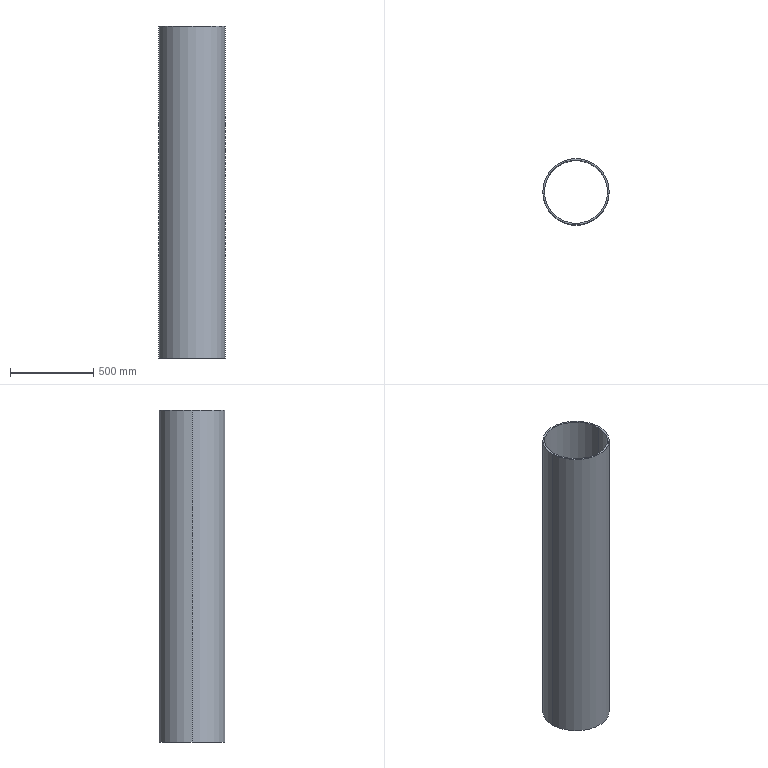Component | SolidWorks | Pipe-1 | 1 solid | 6 faces | box 400 x 400 x 2000 mm | volume 24504423 mm3 | cylinder 4 | plane 2 | commonest cylinder face diameters 380 x2 400 x2
build123d program:
from build123d import *

# Parameters (mm, degrees)
SKETCH1_R           = 200
SKETCH1_R_2         = 190
BOSS_EXTRUDE1_DEPTH = 1000


with BuildPart() as part:
    # Sketch1 → Boss-Extrude1 (new, symmetric)
    with BuildSketch(Plane.XY):
        Circle(SKETCH1_R)
        Circle(SKETCH1_R_2, mode=Mode.SUBTRACT)
    extrude(amount=BOSS_EXTRUDE1_DEPTH, both=True)


solid = part.part
STEP:
#1=CARTESIAN_POINT('',(-7.48,0.,39.37));
#2=VERTEX_POINT('',#1);
#3=CARTESIAN_POINT('',(7.48,0.,39.37));
#4=VERTEX_POINT('',#3);
#5=CARTESIAN_POINT('',(0.,0.,39.37));
#6=DIRECTION('',(0.,0.,1.));
#7=DIRECTION('',(1.,0.,0.));
#8=AXIS2_PLACEMENT_3D('',#5,#6,#7);
#9=CIRCLE('',#8,7.48);
#10=EDGE_CURVE('',#2,#4,#9,.T.);
#11=ORIENTED_EDGE('',*,*,#10,.T.);
#12=CARTESIAN_POINT('',(7.48,0.,-39.37));
#13=VERTEX_POINT('',#12);
#14=CARTESIAN_POINT('',(7.48,0.,39.37));
#15=DIRECTION('',(0.,0.,-1.));
#16=VECTOR('',#15,39.37);
#17=LINE('',#14,#16);
#18=EDGE_CURVE('',#4,#13,#17,.T.);
#19=ORIENTED_EDGE('',*,*,#18,.T.);
#20=CARTESIAN_POINT('',(-7.48,0.,-39.37));
#21=VERTEX_POINT('',#20);
#22=CARTESIAN_POINT('',(0.,0.,-39.37));
#23=DIRECTION('',(0.,0.,1.));
#24=DIRECTION('',(1.,0.,0.));
#25=AXIS2_PLACEMENT_3D('',#22,#23,#24);
#26=CIRCLE('',#25,7.48);
#27=EDGE_CURVE('',#21,#13,#26,.T.);
#28=ORIENTED_EDGE('',*,*,#27,.F.);
#29=CARTESIAN_POINT('',(-7.48,0.,39.37));
#30=DIRECTION('',(0.,0.,-1.));
#31=VECTOR('',#30,39.37);
#32=LINE('',#29,#31);
#33=EDGE_CURVE('',#2,#21,#32,.T.);
#34=ORIENTED_EDGE('',*,*,#33,.F.);
#35=EDGE_LOOP('',(#11,#19,#28,#34));
#36=FACE_OUTER_BOUND('',#35,.T.);
#37=CARTESIAN_POINT('',(0.,0.,39.37));
#38=DIRECTION('',(0.,0.,-1.));
#39=DIRECTION('',(-1.,0.,0.));
#40=AXIS2_PLACEMENT_3D('',#37,#38,#39);
#41=CYLINDRICAL_SURFACE('',#40,7.48);
#42=ADVANCED_FACE('',(#36),#41,.F.);
#43=CARTESIAN_POINT('',(7.874,0.,39.37));
#44=VERTEX_POINT('',#43);
#45=CARTESIAN_POINT('',(-7.874,0.,39.37));
#46=VERTEX_POINT('',#45);
#47=CARTESIAN_POINT('',(0.,0.,39.37));
#48=DIRECTION('',(0.,0.,1.));
#49=DIRECTION('',(1.,0.,0.));
#50=AXIS2_PLACEMENT_3D('',#47,#48,#49);
#51=CIRCLE('',#50,7.874);
#52=EDGE_CURVE('',#44,#46,#51,.T.);
#53=ORIENTED_EDGE('',*,*,#52,.F.);
#54=CARTESIAN_POINT('',(7.874,0.,-39.37));
#55=VERTEX_POINT('',#54);
#56=CARTESIAN_POINT('',(7.874,0.,39.37));
#57=DIRECTION('',(0.,0.,-1.));
#58=VECTOR('',#57,39.37);
#59=LINE('',#56,#58);
#60=EDGE_CURVE('',#44,#55,#59,.T.);
#61=ORIENTED_EDGE('',*,*,#60,.T.);
#62=CARTESIAN_POINT('',(-7.874,0.,-39.37));
#63=VERTEX_POINT('',#62);
#64=CARTESIAN_POINT('',(0.,0.,-39.37));
#65=DIRECTION('',(0.,0.,1.));
#66=DIRECTION('',(1.,0.,0.));
#67=AXIS2_PLACEMENT_3D('',#64,#65,#66);
#68=CIRCLE('',#67,7.874);
#69=EDGE_CURVE('',#55,#63,#68,.T.);
#70=ORIENTED_EDGE('',*,*,#69,.T.);
#71=CARTESIAN_POINT('',(-7.874,0.,39.37));
#72=DIRECTION('',(0.,0.,-1.));
#73=VECTOR('',#72,39.37);
#74=LINE('',#71,#73);
#75=EDGE_CURVE('',#46,#63,#74,.T.);
#76=ORIENTED_EDGE('',*,*,#75,.F.);
#77=EDGE_LOOP('',(#53,#61,#70,#76));
#78=FACE_OUTER_BOUND('',#77,.T.);
#79=CARTESIAN_POINT('',(0.,0.,39.37));
#80=DIRECTION('',(0.,0.,-1.));
#81=DIRECTION('',(-1.,0.,0.));
#82=AXIS2_PLACEMENT_3D('',#79,#80,#81);
#83=CYLINDRICAL_SURFACE('',#82,7.874);
#84=ADVANCED_FACE('',(#78),#83,.T.);
#85=CARTESIAN_POINT('',(0.,0.,39.37));
#86=DIRECTION('',(0.,0.,1.));
#87=DIRECTION('',(1.,0.,0.));
#88=AXIS2_PLACEMENT_3D('',#85,#86,#87);
#89=CIRCLE('',#88,7.874);
#90=EDGE_CURVE('',#46,#44,#89,.T.);
#91=ORIENTED_EDGE('',*,*,#90,.T.);
#92=ORIENTED_EDGE('',*,*,#52,.T.);
#93=EDGE_LOOP('',(#91,#92));
#94=FACE_OUTER_BOUND('',#93,.T.);
#95=ORIENTED_EDGE('',*,*,#10,.F.);
#96=CARTESIAN_POINT('',(0.,0.,39.37));
#97=DIRECTION('',(0.,0.,1.));
#98=DIRECTION('',(1.,0.,0.));
#99=AXIS2_PLACEMENT_3D('',#96,#97,#98);
#100=CIRCLE('',#99,7.48);
#101=EDGE_CURVE('',#4,#2,#100,.T.);
#102=ORIENTED_EDGE('',*,*,#101,.F.);
#103=EDGE_LOOP('',(#95,#102));
#104=FACE_BOUND('',#103,.T.);
#105=CARTESIAN_POINT('',(0.,0.,39.37));
#106=DIRECTION('',(0.,0.,1.));
#107=DIRECTION('',(1.,0.,0.));
#108=AXIS2_PLACEMENT_3D('',#105,#106,#107);
#109=PLANE('',#108);
#110=ADVANCED_FACE('',(#94,#104),#109,.T.);
#111=CARTESIAN_POINT('',(0.,0.,-39.37));
#112=DIRECTION('',(0.,0.,1.));
#113=DIRECTION('',(1.,0.,0.));
#114=AXIS2_PLACEMENT_3D('',#111,#112,#113);
#115=CIRCLE('',#114,7.874);
#116=EDGE_CURVE('',#63,#55,#115,.T.);
#117=ORIENTED_EDGE('',*,*,#116,.F.);
#118=ORIENTED_EDGE('',*,*,#69,.F.);
#119=EDGE_LOOP('',(#117,#118));
#120=FACE_OUTER_BOUND('',#119,.T.);
#121=ORIENTED_EDGE('',*,*,#27,.T.);
#122=CARTESIAN_POINT('',(0.,0.,-39.37));
#123=DIRECTION('',(0.,0.,1.));
#124=DIRECTION('',(1.,0.,0.));
#125=AXIS2_PLACEMENT_3D('',#122,#123,#124);
#126=CIRCLE('',#125,7.48);
#127=EDGE_CURVE('',#13,#21,#126,.T.);
#128=ORIENTED_EDGE('',*,*,#127,.T.);
#129=EDGE_LOOP('',(#121,#128));
#130=FACE_BOUND('',#129,.T.);
#131=CARTESIAN_POINT('',(0.,0.,-39.37));
#132=DIRECTION('',(0.,0.,1.));
#133=DIRECTION('',(1.,0.,0.));
#134=AXIS2_PLACEMENT_3D('',#131,#132,#133);
#135=PLANE('',#134);
#136=ADVANCED_FACE('',(#120,#130),#135,.F.);
#137=ORIENTED_EDGE('',*,*,#60,.F.);
#138=ORIENTED_EDGE('',*,*,#90,.F.);
#139=ORIENTED_EDGE('',*,*,#75,.T.);
#140=ORIENTED_EDGE('',*,*,#116,.T.);
#141=EDGE_LOOP('',(#137,#138,#139,#140));
#142=FACE_OUTER_BOUND('',#141,.T.);
#143=CARTESIAN_POINT('',(0.,0.,39.37));
#144=DIRECTION('',(0.,0.,-1.));
#145=DIRECTION('',(-1.,0.,0.));
#146=AXIS2_PLACEMENT_3D('',#143,#144,#145);
#147=CYLINDRICAL_SURFACE('',#146,7.874);
#148=ADVANCED_FACE('',(#142),#147,.T.);
#149=ORIENTED_EDGE('',*,*,#18,.F.);
#150=ORIENTED_EDGE('',*,*,#101,.T.);
#151=ORIENTED_EDGE('',*,*,#33,.T.);
#152=ORIENTED_EDGE('',*,*,#127,.F.);
#153=EDGE_LOOP('',(#149,#150,#151,#152));
#154=FACE_OUTER_BOUND('',#153,.T.);
#155=CARTESIAN_POINT('',(0.,0.,39.37));
#156=DIRECTION('',(0.,0.,-1.));
#157=DIRECTION('',(-1.,0.,0.));
#158=AXIS2_PLACEMENT_3D('',#155,#156,#157);
#159=CYLINDRICAL_SURFACE('',#158,7.48);
#160=ADVANCED_FACE('',(#154),#159,.F.);
#161=CLOSED_SHELL('',(#42,#84,#110,#136,#148,#160));
#162=MANIFOLD_SOLID_BREP('',#161);
#163=CARTESIAN_POINT('',(0.,0.,0.));
#164=DIRECTION('',(0.,0.,1.));
#165=DIRECTION('',(1.,0.,0.));
#166=AXIS2_PLACEMENT_3D('',#163,#164,#165);
#167=(LENGTH_UNIT()NAMED_UNIT(*)SI_UNIT($,.METRE.));
#168=LENGTH_MEASURE_WITH_UNIT(LENGTH_MEASURE(0.0254),#167);
#169=DIMENSIONAL_EXPONENTS(1.,0.,0.,0.,0.,0.,0.);
#170=(CONVERSION_BASED_UNIT('',#168)LENGTH_UNIT()NAMED_UNIT(#169));
#171=UNCERTAINTY_MEASURE_WITH_UNIT(LENGTH_MEASURE(0.00001),#170,'','');
#172=(NAMED_UNIT(*)PLANE_ANGLE_UNIT()SI_UNIT($,.RADIAN.));
#173=(NAMED_UNIT(*)SI_UNIT($,.STERADIAN.)SOLID_ANGLE_UNIT());
#174=(GEOMETRIC_REPRESENTATION_CONTEXT(3)GLOBAL_UNCERTAINTY_ASSIGNED_CONTEXT((#171))GLOBAL_UNIT_ASSIGNED_CONTEXT((#170,#172,#173))REPRESENTATION_CONTEXT('',''));
#175=ADVANCED_BREP_SHAPE_REPRESENTATION('',(#162,#166),#174);
#176=COLOUR_RGB('',0.7922,0.8196,0.9333);
#177=FILL_AREA_STYLE_COLOUR('',#176);
#178=FILL_AREA_STYLE('',(#177));
#179=SURFACE_STYLE_FILL_AREA(#178);
#180=SURFACE_SIDE_STYLE('',(#179));
#181=SURFACE_STYLE_USAGE(.BOTH.,#180);
#182=PRESENTATION_STYLE_ASSIGNMENT((#181));
#183=STYLED_ITEM('',(#182),#162);
#184=PRESENTATION_LAYER_ASSIGNMENT('','',(#183));
#185=(LENGTH_UNIT()NAMED_UNIT(*)SI_UNIT($,.METRE.));
#186=LENGTH_MEASURE_WITH_UNIT(LENGTH_MEASURE(0.0254),#185);
#187=DIMENSIONAL_EXPONENTS(1.,0.,0.,0.,0.,0.,0.);
#188=(CONVERSION_BASED_UNIT('',#186)LENGTH_UNIT()NAMED_UNIT(#187));
#189=UNCERTAINTY_MEASURE_WITH_UNIT(LENGTH_MEASURE(0.00001),#188,'','');
#190=(NAMED_UNIT(*)PLANE_ANGLE_UNIT()SI_UNIT($,.RADIAN.));
#191=(NAMED_UNIT(*)SI_UNIT($,.STERADIAN.)SOLID_ANGLE_UNIT());
#192=(GEOMETRIC_REPRESENTATION_CONTEXT(3)GLOBAL_UNCERTAINTY_ASSIGNED_CONTEXT((#189))GLOBAL_UNIT_ASSIGNED_CONTEXT((#188,#190,#191))REPRESENTATION_CONTEXT('',''));
#193=MECHANICAL_DESIGN_GEOMETRIC_PRESENTATION_REPRESENTATION('',(#183),#192);